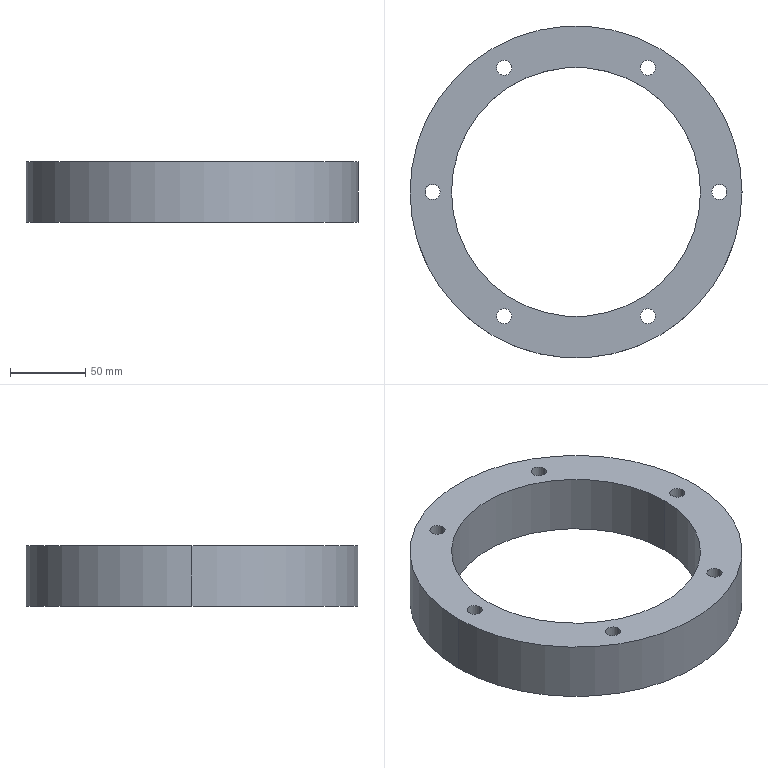Component | SolidWorks | UpperDieHolder-1 | 1 solid | 18 faces | box 220 x 220 x 40 mm | volume 646383 mm3 | cylinder 16 | plane 2 | commonest cylinder face diameters 10 x12 165 x2 220 x2
build123d program:
from build123d import *

# Parameters (mm, degrees)
SKETCH1_R           = 110
SKETCH1_R_2         = 82.5
SKETCH1_R_3         = 5
BOSS_EXTRUDE1_DEPTH = 40


with BuildPart() as part:
    # Sketch1 → Boss-Extrude1 (new body)
    with BuildSketch(Plane.XY):
        Circle(SKETCH1_R)
        Circle(SKETCH1_R_2, mode=Mode.SUBTRACT)
        with Locations((-95, 0)):
            Circle(SKETCH1_R_3, mode=Mode.SUBTRACT)
        with Locations((-47.5, 82.272)):
            Circle(SKETCH1_R_3, mode=Mode.SUBTRACT)
        with Locations((47.5, 82.272)):
            Circle(SKETCH1_R_3, mode=Mode.SUBTRACT)
        with Locations((95, 0)):
            Circle(SKETCH1_R_3, mode=Mode.SUBTRACT)
        with Locations((47.5, -82.272)):
            Circle(SKETCH1_R_3, mode=Mode.SUBTRACT)
        with Locations((-47.5, -82.272)):
            Circle(SKETCH1_R_3, mode=Mode.SUBTRACT)
    extrude(amount=BOSS_EXTRUDE1_DEPTH)


solid = part.part

# Placed as in the assembly
solid = solid.moved(Location((0, 0, -271), (0, 0, 0)))
STEP:
#1=CARTESIAN_POINT('',(-2.067,-3.239,-9.094));
#2=VERTEX_POINT('',#1);
#3=CARTESIAN_POINT('',(-1.673,-3.239,-9.094));
#4=VERTEX_POINT('',#3);
#5=CARTESIAN_POINT('',(-1.87,-3.239,-9.094));
#6=DIRECTION('',(0.,0.,1.));
#7=DIRECTION('',(1.,0.,0.));
#8=AXIS2_PLACEMENT_3D('',#5,#6,#7);
#9=CIRCLE('',#8,0.1969);
#10=EDGE_CURVE('',#2,#4,#9,.T.);
#11=ORIENTED_EDGE('',*,*,#10,.T.);
#12=CARTESIAN_POINT('',(-1.673,-3.239,-10.669));
#13=VERTEX_POINT('',#12);
#14=CARTESIAN_POINT('',(-1.673,-3.239,-9.094));
#15=DIRECTION('',(0.,0.,-1.));
#16=VECTOR('',#15,39.37);
#17=LINE('',#14,#16);
#18=EDGE_CURVE('',#4,#13,#17,.T.);
#19=ORIENTED_EDGE('',*,*,#18,.T.);
#20=CARTESIAN_POINT('',(-2.067,-3.239,-10.669));
#21=VERTEX_POINT('',#20);
#22=CARTESIAN_POINT('',(-1.87,-3.239,-10.669));
#23=DIRECTION('',(0.,0.,1.));
#24=DIRECTION('',(1.,0.,0.));
#25=AXIS2_PLACEMENT_3D('',#22,#23,#24);
#26=CIRCLE('',#25,0.1969);
#27=EDGE_CURVE('',#21,#13,#26,.T.);
#28=ORIENTED_EDGE('',*,*,#27,.F.);
#29=CARTESIAN_POINT('',(-2.067,-3.239,-9.094));
#30=DIRECTION('',(0.,0.,-1.));
#31=VECTOR('',#30,39.37);
#32=LINE('',#29,#31);
#33=EDGE_CURVE('',#2,#21,#32,.T.);
#34=ORIENTED_EDGE('',*,*,#33,.F.);
#35=EDGE_LOOP('',(#11,#19,#28,#34));
#36=FACE_OUTER_BOUND('',#35,.T.);
#37=CARTESIAN_POINT('',(-1.87,-3.239,-9.094));
#38=DIRECTION('',(0.,0.,-1.));
#39=DIRECTION('',(-1.,0.,0.));
#40=AXIS2_PLACEMENT_3D('',#37,#38,#39);
#41=CYLINDRICAL_SURFACE('',#40,0.1969);
#42=ADVANCED_FACE('',(#36),#41,.F.);
#43=CARTESIAN_POINT('',(1.673,-3.239,-9.094));
#44=VERTEX_POINT('',#43);
#45=CARTESIAN_POINT('',(2.067,-3.239,-9.094));
#46=VERTEX_POINT('',#45);
#47=CARTESIAN_POINT('',(1.87,-3.239,-9.094));
#48=DIRECTION('',(0.,0.,1.));
#49=DIRECTION('',(1.,0.,0.));
#50=AXIS2_PLACEMENT_3D('',#47,#48,#49);
#51=CIRCLE('',#50,0.1969);
#52=EDGE_CURVE('',#44,#46,#51,.T.);
#53=ORIENTED_EDGE('',*,*,#52,.T.);
#54=CARTESIAN_POINT('',(2.067,-3.239,-10.669));
#55=VERTEX_POINT('',#54);
#56=CARTESIAN_POINT('',(2.067,-3.239,-9.094));
#57=DIRECTION('',(0.,0.,-1.));
#58=VECTOR('',#57,39.37);
#59=LINE('',#56,#58);
#60=EDGE_CURVE('',#46,#55,#59,.T.);
#61=ORIENTED_EDGE('',*,*,#60,.T.);
#62=CARTESIAN_POINT('',(1.673,-3.239,-10.669));
#63=VERTEX_POINT('',#62);
#64=CARTESIAN_POINT('',(1.87,-3.239,-10.669));
#65=DIRECTION('',(0.,0.,1.));
#66=DIRECTION('',(1.,0.,0.));
#67=AXIS2_PLACEMENT_3D('',#64,#65,#66);
#68=CIRCLE('',#67,0.1969);
#69=EDGE_CURVE('',#63,#55,#68,.T.);
#70=ORIENTED_EDGE('',*,*,#69,.F.);
#71=CARTESIAN_POINT('',(1.673,-3.239,-9.094));
#72=DIRECTION('',(0.,0.,-1.));
#73=VECTOR('',#72,39.37);
#74=LINE('',#71,#73);
#75=EDGE_CURVE('',#44,#63,#74,.T.);
#76=ORIENTED_EDGE('',*,*,#75,.F.);
#77=EDGE_LOOP('',(#53,#61,#70,#76));
#78=FACE_OUTER_BOUND('',#77,.T.);
#79=CARTESIAN_POINT('',(1.87,-3.239,-9.094));
#80=DIRECTION('',(0.,0.,-1.));
#81=DIRECTION('',(-1.,0.,0.));
#82=AXIS2_PLACEMENT_3D('',#79,#80,#81);
#83=CYLINDRICAL_SURFACE('',#82,0.1969);
#84=ADVANCED_FACE('',(#78),#83,.F.);
#85=CARTESIAN_POINT('',(3.543,0.,-9.094));
#86=VERTEX_POINT('',#85);
#87=CARTESIAN_POINT('',(3.937,0.,-9.094));
#88=VERTEX_POINT('',#87);
#89=CARTESIAN_POINT('',(3.74,0.,-9.094));
#90=DIRECTION('',(0.,0.,1.));
#91=DIRECTION('',(1.,0.,0.));
#92=AXIS2_PLACEMENT_3D('',#89,#90,#91);
#93=CIRCLE('',#92,0.1969);
#94=EDGE_CURVE('',#86,#88,#93,.T.);
#95=ORIENTED_EDGE('',*,*,#94,.T.);
#96=CARTESIAN_POINT('',(3.937,0.,-10.669));
#97=VERTEX_POINT('',#96);
#98=CARTESIAN_POINT('',(3.937,0.,-9.094));
#99=DIRECTION('',(0.,0.,-1.));
#100=VECTOR('',#99,39.37);
#101=LINE('',#98,#100);
#102=EDGE_CURVE('',#88,#97,#101,.T.);
#103=ORIENTED_EDGE('',*,*,#102,.T.);
#104=CARTESIAN_POINT('',(3.543,0.,-10.669));
#105=VERTEX_POINT('',#104);
#106=CARTESIAN_POINT('',(3.74,0.,-10.669));
#107=DIRECTION('',(0.,0.,1.));
#108=DIRECTION('',(1.,0.,0.));
#109=AXIS2_PLACEMENT_3D('',#106,#107,#108);
#110=CIRCLE('',#109,0.1969);
#111=EDGE_CURVE('',#105,#97,#110,.T.);
#112=ORIENTED_EDGE('',*,*,#111,.F.);
#113=CARTESIAN_POINT('',(3.543,0.,-9.094));
#114=DIRECTION('',(0.,0.,-1.));
#115=VECTOR('',#114,39.37);
#116=LINE('',#113,#115);
#117=EDGE_CURVE('',#86,#105,#116,.T.);
#118=ORIENTED_EDGE('',*,*,#117,.F.);
#119=EDGE_LOOP('',(#95,#103,#112,#118));
#120=FACE_OUTER_BOUND('',#119,.T.);
#121=CARTESIAN_POINT('',(3.74,0.,-9.094));
#122=DIRECTION('',(0.,0.,-1.));
#123=DIRECTION('',(-1.,0.,0.));
#124=AXIS2_PLACEMENT_3D('',#121,#122,#123);
#125=CYLINDRICAL_SURFACE('',#124,0.1969);
#126=ADVANCED_FACE('',(#120),#125,.F.);
#127=CARTESIAN_POINT('',(1.673,3.239,-9.094));
#128=VERTEX_POINT('',#127);
#129=CARTESIAN_POINT('',(2.067,3.239,-9.094));
#130=VERTEX_POINT('',#129);
#131=CARTESIAN_POINT('',(1.87,3.239,-9.094));
#132=DIRECTION('',(0.,0.,1.));
#133=DIRECTION('',(1.,0.,0.));
#134=AXIS2_PLACEMENT_3D('',#131,#132,#133);
#135=CIRCLE('',#134,0.1969);
#136=EDGE_CURVE('',#128,#130,#135,.T.);
#137=ORIENTED_EDGE('',*,*,#136,.T.);
#138=CARTESIAN_POINT('',(2.067,3.239,-10.669));
#139=VERTEX_POINT('',#138);
#140=CARTESIAN_POINT('',(2.067,3.239,-9.094));
#141=DIRECTION('',(0.,0.,-1.));
#142=VECTOR('',#141,39.37);
#143=LINE('',#140,#142);
#144=EDGE_CURVE('',#130,#139,#143,.T.);
#145=ORIENTED_EDGE('',*,*,#144,.T.);
#146=CARTESIAN_POINT('',(1.673,3.239,-10.669));
#147=VERTEX_POINT('',#146);
#148=CARTESIAN_POINT('',(1.87,3.239,-10.669));
#149=DIRECTION('',(0.,0.,1.));
#150=DIRECTION('',(1.,0.,0.));
#151=AXIS2_PLACEMENT_3D('',#148,#149,#150);
#152=CIRCLE('',#151,0.1969);
#153=EDGE_CURVE('',#147,#139,#152,.T.);
#154=ORIENTED_EDGE('',*,*,#153,.F.);
#155=CARTESIAN_POINT('',(1.673,3.239,-9.094));
#156=DIRECTION('',(0.,0.,-1.));
#157=VECTOR('',#156,39.37);
#158=LINE('',#155,#157);
#159=EDGE_CURVE('',#128,#147,#158,.T.);
#160=ORIENTED_EDGE('',*,*,#159,.F.);
#161=EDGE_LOOP('',(#137,#145,#154,#160));
#162=FACE_OUTER_BOUND('',#161,.T.);
#163=CARTESIAN_POINT('',(1.87,3.239,-9.094));
#164=DIRECTION('',(0.,0.,-1.));
#165=DIRECTION('',(-1.,0.,0.));
#166=AXIS2_PLACEMENT_3D('',#163,#164,#165);
#167=CYLINDRICAL_SURFACE('',#166,0.1969);
#168=ADVANCED_FACE('',(#162),#167,.F.);
#169=CARTESIAN_POINT('',(-2.067,3.239,-9.094));
#170=VERTEX_POINT('',#169);
#171=CARTESIAN_POINT('',(-1.673,3.239,-9.094));
#172=VERTEX_POINT('',#171);
#173=CARTESIAN_POINT('',(-1.87,3.239,-9.094));
#174=DIRECTION('',(0.,0.,1.));
#175=DIRECTION('',(1.,0.,0.));
#176=AXIS2_PLACEMENT_3D('',#173,#174,#175);
#177=CIRCLE('',#176,0.1969);
#178=EDGE_CURVE('',#170,#172,#177,.T.);
#179=ORIENTED_EDGE('',*,*,#178,.T.);
#180=CARTESIAN_POINT('',(-1.673,3.239,-10.669));
#181=VERTEX_POINT('',#180);
#182=CARTESIAN_POINT('',(-1.673,3.239,-9.094));
#183=DIRECTION('',(0.,0.,-1.));
#184=VECTOR('',#183,39.37);
#185=LINE('',#182,#184);
#186=EDGE_CURVE('',#172,#181,#185,.T.);
#187=ORIENTED_EDGE('',*,*,#186,.T.);
#188=CARTESIAN_POINT('',(-2.067,3.239,-10.669));
#189=VERTEX_POINT('',#188);
#190=CARTESIAN_POINT('',(-1.87,3.239,-10.669));
#191=DIRECTION('',(0.,0.,1.));
#192=DIRECTION('',(1.,0.,0.));
#193=AXIS2_PLACEMENT_3D('',#190,#191,#192);
#194=CIRCLE('',#193,0.1969);
#195=EDGE_CURVE('',#189,#181,#194,.T.);
#196=ORIENTED_EDGE('',*,*,#195,.F.);
#197=CARTESIAN_POINT('',(-2.067,3.239,-9.094));
#198=DIRECTION('',(0.,0.,-1.));
#199=VECTOR('',#198,39.37);
#200=LINE('',#197,#199);
#201=EDGE_CURVE('',#170,#189,#200,.T.);
#202=ORIENTED_EDGE('',*,*,#201,.F.);
#203=EDGE_LOOP('',(#179,#187,#196,#202));
#204=FACE_OUTER_BOUND('',#203,.T.);
#205=CARTESIAN_POINT('',(-1.87,3.239,-9.094));
#206=DIRECTION('',(0.,0.,-1.));
#207=DIRECTION('',(-1.,0.,0.));
#208=AXIS2_PLACEMENT_3D('',#205,#206,#207);
#209=CYLINDRICAL_SURFACE('',#208,0.1969);
#210=ADVANCED_FACE('',(#204),#209,.F.);
#211=CARTESIAN_POINT('',(-3.937,0.,-9.094));
#212=VERTEX_POINT('',#211);
#213=CARTESIAN_POINT('',(-3.543,0.,-9.094));
#214=VERTEX_POINT('',#213);
#215=CARTESIAN_POINT('',(-3.74,0.,-9.094));
#216=DIRECTION('',(0.,0.,1.));
#217=DIRECTION('',(1.,0.,0.));
#218=AXIS2_PLACEMENT_3D('',#215,#216,#217);
#219=CIRCLE('',#218,0.1969);
#220=EDGE_CURVE('',#212,#214,#219,.T.);
#221=ORIENTED_EDGE('',*,*,#220,.T.);
#222=CARTESIAN_POINT('',(-3.543,0.,-10.669));
#223=VERTEX_POINT('',#222);
#224=CARTESIAN_POINT('',(-3.543,0.,-9.094));
#225=DIRECTION('',(0.,0.,-1.));
#226=VECTOR('',#225,39.37);
#227=LINE('',#224,#226);
#228=EDGE_CURVE('',#214,#223,#227,.T.);
#229=ORIENTED_EDGE('',*,*,#228,.T.);
#230=CARTESIAN_POINT('',(-3.937,0.,-10.669));
#231=VERTEX_POINT('',#230);
#232=CARTESIAN_POINT('',(-3.74,0.,-10.669));
#233=DIRECTION('',(0.,0.,1.));
#234=DIRECTION('',(1.,0.,0.));
#235=AXIS2_PLACEMENT_3D('',#232,#233,#234);
#236=CIRCLE('',#235,0.1969);
#237=EDGE_CURVE('',#231,#223,#236,.T.);
#238=ORIENTED_EDGE('',*,*,#237,.F.);
#239=CARTESIAN_POINT('',(-3.937,0.,-9.094));
#240=DIRECTION('',(0.,0.,-1.));
#241=VECTOR('',#240,39.37);
#242=LINE('',#239,#241);
#243=EDGE_CURVE('',#212,#231,#242,.T.);
#244=ORIENTED_EDGE('',*,*,#243,.F.);
#245=EDGE_LOOP('',(#221,#229,#238,#244));
#246=FACE_OUTER_BOUND('',#245,.T.);
#247=CARTESIAN_POINT('',(-3.74,0.,-9.094));
#248=DIRECTION('',(0.,0.,-1.));
#249=DIRECTION('',(-1.,0.,0.));
#250=AXIS2_PLACEMENT_3D('',#247,#248,#249);
#251=CYLINDRICAL_SURFACE('',#250,0.1969);
#252=ADVANCED_FACE('',(#246),#251,.F.);
#253=CARTESIAN_POINT('',(-3.248,0.,-9.094));
#254=VERTEX_POINT('',#253);
#255=CARTESIAN_POINT('',(3.248,0.,-9.094));
#256=VERTEX_POINT('',#255);
#257=CARTESIAN_POINT('',(-0.,0.,-9.094));
#258=DIRECTION('',(0.,0.,1.));
#259=DIRECTION('',(1.,0.,0.));
#260=AXIS2_PLACEMENT_3D('',#257,#258,#259);
#261=CIRCLE('',#260,3.248);
#262=EDGE_CURVE('',#254,#256,#261,.T.);
#263=ORIENTED_EDGE('',*,*,#262,.T.);
#264=CARTESIAN_POINT('',(3.248,0.,-10.669));
#265=VERTEX_POINT('',#264);
#266=CARTESIAN_POINT('',(3.248,0.,-9.094));
#267=DIRECTION('',(0.,0.,-1.));
#268=VECTOR('',#267,39.37);
#269=LINE('',#266,#268);
#270=EDGE_CURVE('',#256,#265,#269,.T.);
#271=ORIENTED_EDGE('',*,*,#270,.T.);
#272=CARTESIAN_POINT('',(-3.248,0.,-10.669));
#273=VERTEX_POINT('',#272);
#274=CARTESIAN_POINT('',(-0.,0.,-10.669));
#275=DIRECTION('',(0.,0.,1.));
#276=DIRECTION('',(1.,0.,0.));
#277=AXIS2_PLACEMENT_3D('',#274,#275,#276);
#278=CIRCLE('',#277,3.248);
#279=EDGE_CURVE('',#273,#265,#278,.T.);
#280=ORIENTED_EDGE('',*,*,#279,.F.);
#281=CARTESIAN_POINT('',(-3.248,0.,-9.094));
#282=DIRECTION('',(0.,0.,-1.));
#283=VECTOR('',#282,39.37);
#284=LINE('',#281,#283);
#285=EDGE_CURVE('',#254,#273,#284,.T.);
#286=ORIENTED_EDGE('',*,*,#285,.F.);
#287=EDGE_LOOP('',(#263,#271,#280,#286));
#288=FACE_OUTER_BOUND('',#287,.T.);
#289=CARTESIAN_POINT('',(-0.,0.,-9.094));
#290=DIRECTION('',(0.,0.,-1.));
#291=DIRECTION('',(-1.,0.,0.));
#292=AXIS2_PLACEMENT_3D('',#289,#290,#291);
#293=CYLINDRICAL_SURFACE('',#292,3.248);
#294=ADVANCED_FACE('',(#288),#293,.F.);
#295=CARTESIAN_POINT('',(4.331,0.,-9.094));
#296=VERTEX_POINT('',#295);
#297=CARTESIAN_POINT('',(-4.331,0.,-9.094));
#298=VERTEX_POINT('',#297);
#299=CARTESIAN_POINT('',(-0.,0.,-9.094));
#300=DIRECTION('',(0.,0.,1.));
#301=DIRECTION('',(1.,0.,0.));
#302=AXIS2_PLACEMENT_3D('',#299,#300,#301);
#303=CIRCLE('',#302,4.331);
#304=EDGE_CURVE('',#296,#298,#303,.T.);
#305=ORIENTED_EDGE('',*,*,#304,.F.);
#306=CARTESIAN_POINT('',(4.331,0.,-10.669));
#307=VERTEX_POINT('',#306);
#308=CARTESIAN_POINT('',(4.331,0.,-9.094));
#309=DIRECTION('',(0.,0.,-1.));
#310=VECTOR('',#309,39.37);
#311=LINE('',#308,#310);
#312=EDGE_CURVE('',#296,#307,#311,.T.);
#313=ORIENTED_EDGE('',*,*,#312,.T.);
#314=CARTESIAN_POINT('',(-4.331,0.,-10.669));
#315=VERTEX_POINT('',#314);
#316=CARTESIAN_POINT('',(-0.,0.,-10.669));
#317=DIRECTION('',(0.,0.,1.));
#318=DIRECTION('',(1.,0.,0.));
#319=AXIS2_PLACEMENT_3D('',#316,#317,#318);
#320=CIRCLE('',#319,4.331);
#321=EDGE_CURVE('',#307,#315,#320,.T.);
#322=ORIENTED_EDGE('',*,*,#321,.T.);
#323=CARTESIAN_POINT('',(-4.331,0.,-9.094));
#324=DIRECTION('',(0.,0.,-1.));
#325=VECTOR('',#324,39.37);
#326=LINE('',#323,#325);
#327=EDGE_CURVE('',#298,#315,#326,.T.);
#328=ORIENTED_EDGE('',*,*,#327,.F.);
#329=EDGE_LOOP('',(#305,#313,#322,#328));
#330=FACE_OUTER_BOUND('',#329,.T.);
#331=CARTESIAN_POINT('',(-0.,0.,-9.094));
#332=DIRECTION('',(0.,0.,-1.));
#333=DIRECTION('',(-1.,0.,0.));
#334=AXIS2_PLACEMENT_3D('',#331,#332,#333);
#335=CYLINDRICAL_SURFACE('',#334,4.331);
#336=ADVANCED_FACE('',(#330),#335,.T.);
#337=ORIENTED_EDGE('',*,*,#52,.F.);
#338=CARTESIAN_POINT('',(1.87,-3.239,-9.094));
#339=DIRECTION('',(0.,0.,1.));
#340=DIRECTION('',(1.,0.,0.));
#341=AXIS2_PLACEMENT_3D('',#338,#339,#340);
#342=CIRCLE('',#341,0.1969);
#343=EDGE_CURVE('',#46,#44,#342,.T.);
#344=ORIENTED_EDGE('',*,*,#343,.F.);
#345=EDGE_LOOP('',(#337,#344));
#346=FACE_BOUND('',#345,.T.);
#347=ORIENTED_EDGE('',*,*,#136,.F.);
#348=CARTESIAN_POINT('',(1.87,3.239,-9.094));
#349=DIRECTION('',(0.,0.,1.));
#350=DIRECTION('',(1.,0.,0.));
#351=AXIS2_PLACEMENT_3D('',#348,#349,#350);
#352=CIRCLE('',#351,0.1969);
#353=EDGE_CURVE('',#130,#128,#352,.T.);
#354=ORIENTED_EDGE('',*,*,#353,.F.);
#355=EDGE_LOOP('',(#347,#354));
#356=FACE_BOUND('',#355,.T.);
#357=ORIENTED_EDGE('',*,*,#220,.F.);
#358=CARTESIAN_POINT('',(-3.74,0.,-9.094));
#359=DIRECTION('',(0.,0.,1.));
#360=DIRECTION('',(1.,0.,0.));
#361=AXIS2_PLACEMENT_3D('',#358,#359,#360);
#362=CIRCLE('',#361,0.1969);
#363=EDGE_CURVE('',#214,#212,#362,.T.);
#364=ORIENTED_EDGE('',*,*,#363,.F.);
#365=EDGE_LOOP('',(#357,#364));
#366=FACE_BOUND('',#365,.T.);
#367=CARTESIAN_POINT('',(-0.,0.,-9.094));
#368=DIRECTION('',(0.,0.,1.));
#369=DIRECTION('',(1.,0.,0.));
#370=AXIS2_PLACEMENT_3D('',#367,#368,#369);
#371=CIRCLE('',#370,4.331);
#372=EDGE_CURVE('',#298,#296,#371,.T.);
#373=ORIENTED_EDGE('',*,*,#372,.T.);
#374=ORIENTED_EDGE('',*,*,#304,.T.);
#375=EDGE_LOOP('',(#373,#374));
#376=FACE_OUTER_BOUND('',#375,.T.);
#377=ORIENTED_EDGE('',*,*,#262,.F.);
#378=CARTESIAN_POINT('',(-0.,0.,-9.094));
#379=DIRECTION('',(0.,0.,1.));
#380=DIRECTION('',(1.,0.,0.));
#381=AXIS2_PLACEMENT_3D('',#378,#379,#380);
#382=CIRCLE('',#381,3.248);
#383=EDGE_CURVE('',#256,#254,#382,.T.);
#384=ORIENTED_EDGE('',*,*,#383,.F.);
#385=EDGE_LOOP('',(#377,#384));
#386=FACE_BOUND('',#385,.T.);
#387=ORIENTED_EDGE('',*,*,#178,.F.);
#388=CARTESIAN_POINT('',(-1.87,3.239,-9.094));
#389=DIRECTION('',(0.,0.,1.));
#390=DIRECTION('',(1.,0.,0.));
#391=AXIS2_PLACEMENT_3D('',#388,#389,#390);
#392=CIRCLE('',#391,0.1969);
#393=EDGE_CURVE('',#172,#170,#392,.T.);
#394=ORIENTED_EDGE('',*,*,#393,.F.);
#395=EDGE_LOOP('',(#387,#394));
#396=FACE_BOUND('',#395,.T.);
#397=ORIENTED_EDGE('',*,*,#94,.F.);
#398=CARTESIAN_POINT('',(3.74,0.,-9.094));
#399=DIRECTION('',(0.,0.,1.));
#400=DIRECTION('',(1.,0.,0.));
#401=AXIS2_PLACEMENT_3D('',#398,#399,#400);
#402=CIRCLE('',#401,0.1969);
#403=EDGE_CURVE('',#88,#86,#402,.T.);
#404=ORIENTED_EDGE('',*,*,#403,.F.);
#405=EDGE_LOOP('',(#397,#404));
#406=FACE_BOUND('',#405,.T.);
#407=ORIENTED_EDGE('',*,*,#10,.F.);
#408=CARTESIAN_POINT('',(-1.87,-3.239,-9.094));
#409=DIRECTION('',(0.,0.,1.));
#410=DIRECTION('',(1.,0.,0.));
#411=AXIS2_PLACEMENT_3D('',#408,#409,#410);
#412=CIRCLE('',#411,0.1969);
#413=EDGE_CURVE('',#4,#2,#412,.T.);
#414=ORIENTED_EDGE('',*,*,#413,.F.);
#415=EDGE_LOOP('',(#407,#414));
#416=FACE_BOUND('',#415,.T.);
#417=CARTESIAN_POINT('',(-0.,0.,-9.094));
#418=DIRECTION('',(0.,0.,1.));
#419=DIRECTION('',(1.,0.,0.));
#420=AXIS2_PLACEMENT_3D('',#417,#418,#419);
#421=PLANE('',#420);
#422=ADVANCED_FACE('',(#346,#356,#366,#376,#386,#396,#406,#416),#421,.T.);
#423=CARTESIAN_POINT('',(-0.,0.,-10.669));
#424=DIRECTION('',(0.,0.,1.));
#425=DIRECTION('',(1.,0.,0.));
#426=AXIS2_PLACEMENT_3D('',#423,#424,#425);
#427=CIRCLE('',#426,4.331);
#428=EDGE_CURVE('',#315,#307,#427,.T.);
#429=ORIENTED_EDGE('',*,*,#428,.F.);
#430=ORIENTED_EDGE('',*,*,#321,.F.);
#431=EDGE_LOOP('',(#429,#430));
#432=FACE_OUTER_BOUND('',#431,.T.);
#433=ORIENTED_EDGE('',*,*,#279,.T.);
#434=CARTESIAN_POINT('',(-0.,0.,-10.669));
#435=DIRECTION('',(0.,0.,1.));
#436=DIRECTION('',(1.,0.,0.));
#437=AXIS2_PLACEMENT_3D('',#434,#435,#436);
#438=CIRCLE('',#437,3.248);
#439=EDGE_CURVE('',#265,#273,#438,.T.);
#440=ORIENTED_EDGE('',*,*,#439,.T.);
#441=EDGE_LOOP('',(#433,#440));
#442=FACE_BOUND('',#441,.T.);
#443=ORIENTED_EDGE('',*,*,#237,.T.);
#444=CARTESIAN_POINT('',(-3.74,0.,-10.669));
#445=DIRECTION('',(0.,0.,1.));
#446=DIRECTION('',(1.,0.,0.));
#447=AXIS2_PLACEMENT_3D('',#444,#445,#446);
#448=CIRCLE('',#447,0.1969);
#449=EDGE_CURVE('',#223,#231,#448,.T.);
#450=ORIENTED_EDGE('',*,*,#449,.T.);
#451=EDGE_LOOP('',(#443,#450));
#452=FACE_BOUND('',#451,.T.);
#453=ORIENTED_EDGE('',*,*,#195,.T.);
#454=CARTESIAN_POINT('',(-1.87,3.239,-10.669));
#455=DIRECTION('',(0.,0.,1.));
#456=DIRECTION('',(1.,0.,0.));
#457=AXIS2_PLACEMENT_3D('',#454,#455,#456);
#458=CIRCLE('',#457,0.1969);
#459=EDGE_CURVE('',#181,#189,#458,.T.);
#460=ORIENTED_EDGE('',*,*,#459,.T.);
#461=EDGE_LOOP('',(#453,#460));
#462=FACE_BOUND('',#461,.T.);
#463=ORIENTED_EDGE('',*,*,#153,.T.);
#464=CARTESIAN_POINT('',(1.87,3.239,-10.669));
#465=DIRECTION('',(0.,0.,1.));
#466=DIRECTION('',(1.,0.,0.));
#467=AXIS2_PLACEMENT_3D('',#464,#465,#466);
#468=CIRCLE('',#467,0.1969);
#469=EDGE_CURVE('',#139,#147,#468,.T.);
#470=ORIENTED_EDGE('',*,*,#469,.T.);
#471=EDGE_LOOP('',(#463,#470));
#472=FACE_BOUND('',#471,.T.);
#473=ORIENTED_EDGE('',*,*,#111,.T.);
#474=CARTESIAN_POINT('',(3.74,0.,-10.669));
#475=DIRECTION('',(0.,0.,1.));
#476=DIRECTION('',(1.,0.,0.));
#477=AXIS2_PLACEMENT_3D('',#474,#475,#476);
#478=CIRCLE('',#477,0.1969);
#479=EDGE_CURVE('',#97,#105,#478,.T.);
#480=ORIENTED_EDGE('',*,*,#479,.T.);
#481=EDGE_LOOP('',(#473,#480));
#482=FACE_BOUND('',#481,.T.);
#483=ORIENTED_EDGE('',*,*,#69,.T.);
#484=CARTESIAN_POINT('',(1.87,-3.239,-10.669));
#485=DIRECTION('',(0.,0.,1.));
#486=DIRECTION('',(1.,0.,0.));
#487=AXIS2_PLACEMENT_3D('',#484,#485,#486);
#488=CIRCLE('',#487,0.1969);
#489=EDGE_CURVE('',#55,#63,#488,.T.);
#490=ORIENTED_EDGE('',*,*,#489,.T.);
#491=EDGE_LOOP('',(#483,#490));
#492=FACE_BOUND('',#491,.T.);
#493=ORIENTED_EDGE('',*,*,#27,.T.);
#494=CARTESIAN_POINT('',(-1.87,-3.239,-10.669));
#495=DIRECTION('',(0.,0.,1.));
#496=DIRECTION('',(1.,0.,0.));
#497=AXIS2_PLACEMENT_3D('',#494,#495,#496);
#498=CIRCLE('',#497,0.1969);
#499=EDGE_CURVE('',#13,#21,#498,.T.);
#500=ORIENTED_EDGE('',*,*,#499,.T.);
#501=EDGE_LOOP('',(#493,#500));
#502=FACE_BOUND('',#501,.T.);
#503=CARTESIAN_POINT('',(-0.,0.,-10.669));
#504=DIRECTION('',(0.,0.,1.));
#505=DIRECTION('',(1.,0.,0.));
#506=AXIS2_PLACEMENT_3D('',#503,#504,#505);
#507=PLANE('',#506);
#508=ADVANCED_FACE('',(#432,#442,#452,#462,#472,#482,#492,#502),#507,.F.);
#509=ORIENTED_EDGE('',*,*,#312,.F.);
#510=ORIENTED_EDGE('',*,*,#372,.F.);
#511=ORIENTED_EDGE('',*,*,#327,.T.);
#512=ORIENTED_EDGE('',*,*,#428,.T.);
#513=EDGE_LOOP('',(#509,#510,#511,#512));
#514=FACE_OUTER_BOUND('',#513,.T.);
#515=CARTESIAN_POINT('',(-0.,0.,-9.094));
#516=DIRECTION('',(0.,0.,-1.));
#517=DIRECTION('',(-1.,0.,0.));
#518=AXIS2_PLACEMENT_3D('',#515,#516,#517);
#519=CYLINDRICAL_SURFACE('',#518,4.331);
#520=ADVANCED_FACE('',(#514),#519,.T.);
#521=ORIENTED_EDGE('',*,*,#270,.F.);
#522=ORIENTED_EDGE('',*,*,#383,.T.);
#523=ORIENTED_EDGE('',*,*,#285,.T.);
#524=ORIENTED_EDGE('',*,*,#439,.F.);
#525=EDGE_LOOP('',(#521,#522,#523,#524));
#526=FACE_OUTER_BOUND('',#525,.T.);
#527=CARTESIAN_POINT('',(-0.,0.,-9.094));
#528=DIRECTION('',(0.,0.,-1.));
#529=DIRECTION('',(-1.,0.,0.));
#530=AXIS2_PLACEMENT_3D('',#527,#528,#529);
#531=CYLINDRICAL_SURFACE('',#530,3.248);
#532=ADVANCED_FACE('',(#526),#531,.F.);
#533=ORIENTED_EDGE('',*,*,#228,.F.);
#534=ORIENTED_EDGE('',*,*,#363,.T.);
#535=ORIENTED_EDGE('',*,*,#243,.T.);
#536=ORIENTED_EDGE('',*,*,#449,.F.);
#537=EDGE_LOOP('',(#533,#534,#535,#536));
#538=FACE_OUTER_BOUND('',#537,.T.);
#539=CARTESIAN_POINT('',(-3.74,0.,-9.094));
#540=DIRECTION('',(0.,0.,-1.));
#541=DIRECTION('',(-1.,0.,0.));
#542=AXIS2_PLACEMENT_3D('',#539,#540,#541);
#543=CYLINDRICAL_SURFACE('',#542,0.1969);
#544=ADVANCED_FACE('',(#538),#543,.F.);
#545=ORIENTED_EDGE('',*,*,#186,.F.);
#546=ORIENTED_EDGE('',*,*,#393,.T.);
#547=ORIENTED_EDGE('',*,*,#201,.T.);
#548=ORIENTED_EDGE('',*,*,#459,.F.);
#549=EDGE_LOOP('',(#545,#546,#547,#548));
#550=FACE_OUTER_BOUND('',#549,.T.);
#551=CARTESIAN_POINT('',(-1.87,3.239,-9.094));
#552=DIRECTION('',(0.,0.,-1.));
#553=DIRECTION('',(-1.,0.,0.));
#554=AXIS2_PLACEMENT_3D('',#551,#552,#553);
#555=CYLINDRICAL_SURFACE('',#554,0.1969);
#556=ADVANCED_FACE('',(#550),#555,.F.);
#557=ORIENTED_EDGE('',*,*,#144,.F.);
#558=ORIENTED_EDGE('',*,*,#353,.T.);
#559=ORIENTED_EDGE('',*,*,#159,.T.);
#560=ORIENTED_EDGE('',*,*,#469,.F.);
#561=EDGE_LOOP('',(#557,#558,#559,#560));
#562=FACE_OUTER_BOUND('',#561,.T.);
#563=CARTESIAN_POINT('',(1.87,3.239,-9.094));
#564=DIRECTION('',(0.,0.,-1.));
#565=DIRECTION('',(-1.,0.,0.));
#566=AXIS2_PLACEMENT_3D('',#563,#564,#565);
#567=CYLINDRICAL_SURFACE('',#566,0.1969);
#568=ADVANCED_FACE('',(#562),#567,.F.);
#569=ORIENTED_EDGE('',*,*,#102,.F.);
#570=ORIENTED_EDGE('',*,*,#403,.T.);
#571=ORIENTED_EDGE('',*,*,#117,.T.);
#572=ORIENTED_EDGE('',*,*,#479,.F.);
#573=EDGE_LOOP('',(#569,#570,#571,#572));
#574=FACE_OUTER_BOUND('',#573,.T.);
#575=CARTESIAN_POINT('',(3.74,0.,-9.094));
#576=DIRECTION('',(0.,0.,-1.));
#577=DIRECTION('',(-1.,0.,0.));
#578=AXIS2_PLACEMENT_3D('',#575,#576,#577);
#579=CYLINDRICAL_SURFACE('',#578,0.1969);
#580=ADVANCED_FACE('',(#574),#579,.F.);
#581=ORIENTED_EDGE('',*,*,#60,.F.);
#582=ORIENTED_EDGE('',*,*,#343,.T.);
#583=ORIENTED_EDGE('',*,*,#75,.T.);
#584=ORIENTED_EDGE('',*,*,#489,.F.);
#585=EDGE_LOOP('',(#581,#582,#583,#584));
#586=FACE_OUTER_BOUND('',#585,.T.);
#587=CARTESIAN_POINT('',(1.87,-3.239,-9.094));
#588=DIRECTION('',(0.,0.,-1.));
#589=DIRECTION('',(-1.,0.,0.));
#590=AXIS2_PLACEMENT_3D('',#587,#588,#589);
#591=CYLINDRICAL_SURFACE('',#590,0.1969);
#592=ADVANCED_FACE('',(#586),#591,.F.);
#593=ORIENTED_EDGE('',*,*,#18,.F.);
#594=ORIENTED_EDGE('',*,*,#413,.T.);
#595=ORIENTED_EDGE('',*,*,#33,.T.);
#596=ORIENTED_EDGE('',*,*,#499,.F.);
#597=EDGE_LOOP('',(#593,#594,#595,#596));
#598=FACE_OUTER_BOUND('',#597,.T.);
#599=CARTESIAN_POINT('',(-1.87,-3.239,-9.094));
#600=DIRECTION('',(0.,0.,-1.));
#601=DIRECTION('',(-1.,0.,0.));
#602=AXIS2_PLACEMENT_3D('',#599,#600,#601);
#603=CYLINDRICAL_SURFACE('',#602,0.1969);
#604=ADVANCED_FACE('',(#598),#603,.F.);
#605=CLOSED_SHELL('',(#42,#84,#126,#168,#210,#252,#294,#336,#422,#508,#520,#532,#544,#556,#568,#580,#592,#604));
#606=MANIFOLD_SOLID_BREP('',#605);
#607=CARTESIAN_POINT('',(0.,0.,0.));
#608=DIRECTION('',(0.,0.,1.));
#609=DIRECTION('',(1.,0.,0.));
#610=AXIS2_PLACEMENT_3D('',#607,#608,#609);
#611=(LENGTH_UNIT()NAMED_UNIT(*)SI_UNIT($,.METRE.));
#612=LENGTH_MEASURE_WITH_UNIT(LENGTH_MEASURE(0.0254),#611);
#613=DIMENSIONAL_EXPONENTS(1.,0.,0.,0.,0.,0.,0.);
#614=(CONVERSION_BASED_UNIT('',#612)LENGTH_UNIT()NAMED_UNIT(#613));
#615=UNCERTAINTY_MEASURE_WITH_UNIT(LENGTH_MEASURE(0.00001),#614,'','');
#616=(NAMED_UNIT(*)PLANE_ANGLE_UNIT()SI_UNIT($,.RADIAN.));
#617=(NAMED_UNIT(*)SI_UNIT($,.STERADIAN.)SOLID_ANGLE_UNIT());
#618=(GEOMETRIC_REPRESENTATION_CONTEXT(3)GLOBAL_UNCERTAINTY_ASSIGNED_CONTEXT((#615))GLOBAL_UNIT_ASSIGNED_CONTEXT((#614,#616,#617))REPRESENTATION_CONTEXT('',''));
#619=ADVANCED_BREP_SHAPE_REPRESENTATION('',(#606,#610),#618);
#620=COLOUR_RGB('',0.7922,0.8196,0.9333);
#621=FILL_AREA_STYLE_COLOUR('',#620);
#622=FILL_AREA_STYLE('',(#621));
#623=SURFACE_STYLE_FILL_AREA(#622);
#624=SURFACE_SIDE_STYLE('',(#623));
#625=SURFACE_STYLE_USAGE(.BOTH.,#624);
#626=PRESENTATION_STYLE_ASSIGNMENT((#625));
#627=STYLED_ITEM('',(#626),#606);
#628=(LENGTH_UNIT()NAMED_UNIT(*)SI_UNIT($,.METRE.));
#629=LENGTH_MEASURE_WITH_UNIT(LENGTH_MEASURE(0.0254),#628);
#630=DIMENSIONAL_EXPONENTS(1.,0.,0.,0.,0.,0.,0.);
#631=(CONVERSION_BASED_UNIT('',#629)LENGTH_UNIT()NAMED_UNIT(#630));
#632=UNCERTAINTY_MEASURE_WITH_UNIT(LENGTH_MEASURE(0.00001),#631,'','');
#633=(NAMED_UNIT(*)PLANE_ANGLE_UNIT()SI_UNIT($,.RADIAN.));
#634=(NAMED_UNIT(*)SI_UNIT($,.STERADIAN.)SOLID_ANGLE_UNIT());
#635=(GEOMETRIC_REPRESENTATION_CONTEXT(3)GLOBAL_UNCERTAINTY_ASSIGNED_CONTEXT((#632))GLOBAL_UNIT_ASSIGNED_CONTEXT((#631,#633,#634))REPRESENTATION_CONTEXT('',''));
#636=MECHANICAL_DESIGN_GEOMETRIC_PRESENTATION_REPRESENTATION('',(#627),#635);
#637=PRESENTATION_LAYER_ASSIGNMENT('','',(#627));